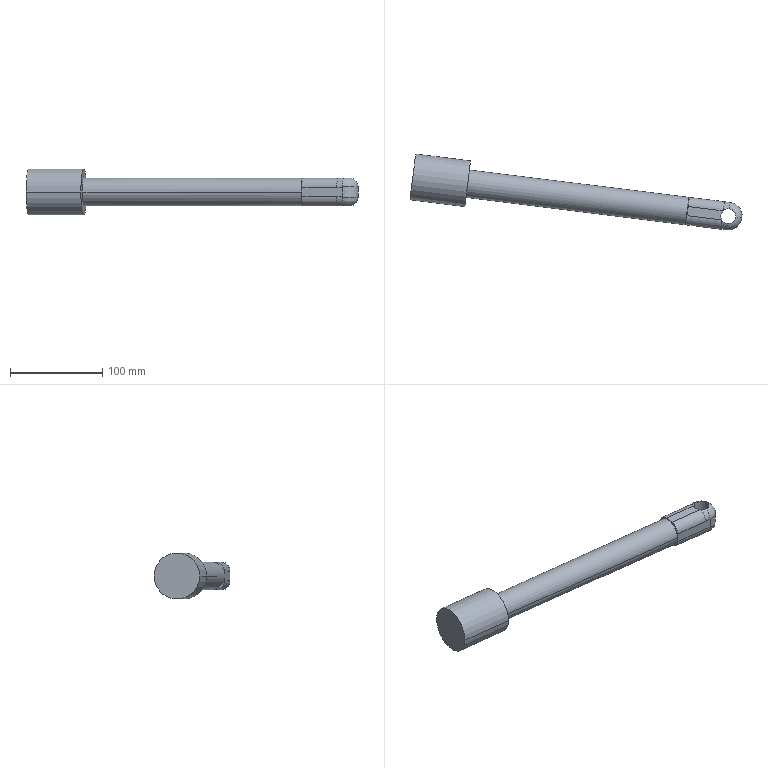Component | SolidWorks | Piston2-1 | 1 solid | 49 faces | volume 327244 mm3 | cylinder 19 | spline 12 | plane 10 | torus 8 | commonest cylinder face diameters 1 x8 20 x4 30 x3 16 x2 50 x2